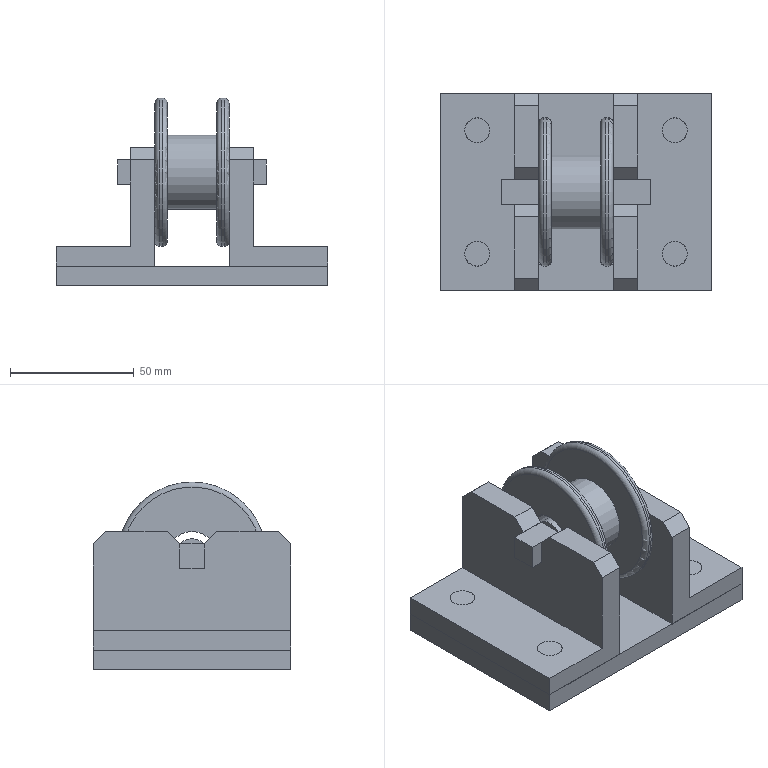Assembly | NX | mm | 9 component files | 9 solids | 105 faces | box 110 x 80 x 76 mm | volume 220983 mm3 | plane 76 | cylinder 25 | torus 4 | commonest cylinder face diameters 6 x12 10 x8 60 x2 30 x1 20 x1 14.142 x1
Bill of materials:
unnamed part 1 | 2 |  | L-shaped bracket: a flat rectangular base flange with an upright wall along one long edge. The wall has chamfered top outer corners and a central rectangular notch cut down from its top edge. The base has two holes.
unnamed part 2 | 4 |  | Headed cylindrical pin: a short, thin round head (flange) on top of a smaller-diameter straight cylindrical shank.
unnamed part 3 | 1 |  | Spool/bobbin shape: two equal round flanges with rounded rims, joined by a central cylindrical hub, with a through bore along the axis.
unnamed part 4 | 1 |  | Flat rectangular plate with four round through-holes, one near each corner, laid out in a rectangle.
unnamed part 5 | 1 |  | Straight square-section bar with a larger-diameter coaxial cylindrical section in the middle of its length, so the square ends stick out from both sides of the cylinder.
Mates:
1. fix | 5 1 component
2. concentric | 3 2 edge | 5 1 edge
3. concentric | 3 2 edge | 5 1 edge
4. concentric | 3 1 edge | 5 1 edge
5. concentric | 3 1 edge | 5 1 edge
6. center | 4 1 face | 4 1 face | 3 1 face | 3 2 face
7. touch align | 4 1 face | 3 1 face
8. center | 4 1 face | 4 1 face | 3 1 face | 3 1 face
9. center | 2 1 face | 2 1 face | 4 1 face | 4 1 face
10. touch align | 2 1 face | 4 1 face
11. concentric | 1 4 edge | 3 2 edge
12. concentric | 1 3 edge | 3 2 edge
13. concentric | 1 2 edge | 3 1 edge
14. concentric | 1 1 edge | 3 1 edge